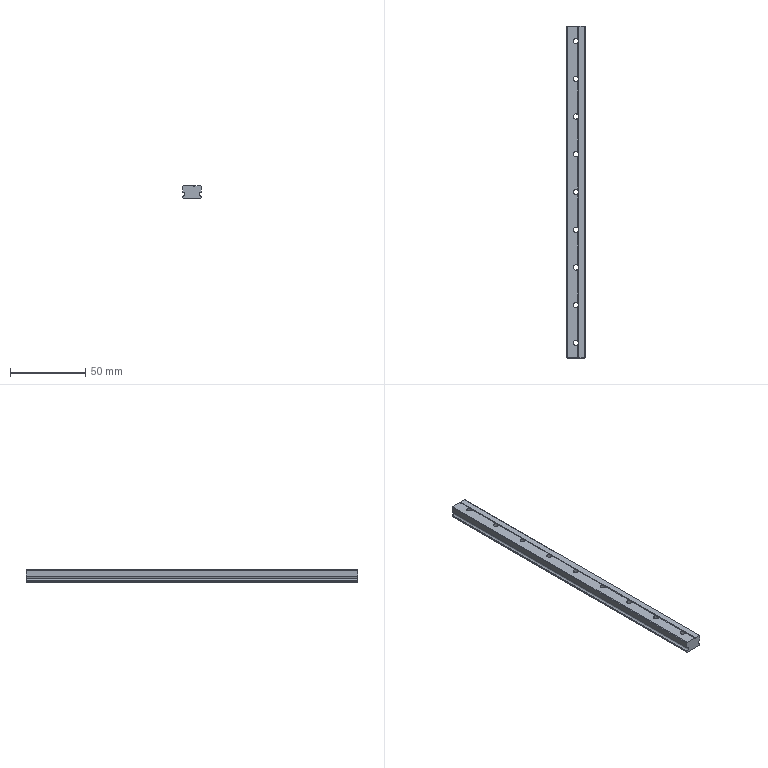Component | SolidWorks | LinearGuideMGN12(HIWIN)-1 | 1 solid | 169 faces | box 12 x 220 x 8 mm | volume 18690 mm3 | plane 114 | cylinder 40 | spline 15 | commonest cylinder face diameters 6 x18 3.5 x18 2.5 x3 0.6 x1 | material Chrome Stainless Steel
build123d program:
from build123d import *

# Parameters (mm, degrees)
BOSS_EXTRUDE1_DEPTH                             = 220
M3_HEX_SOCKET_HEAD_CAP_SCREW_CBORE1_D           = 3.5
M3_HEX_SOCKET_HEAD_CAP_SCREW_CBORE1_CBORE_D     = 6
M3_HEX_SOCKET_HEAD_CAP_SCREW_CBORE1_CBORE_DEPTH = 3.5
LPATTERN1_COUNT                                 = 9
LPATTERN1_PITCH                                 = 25
SKETCH6_W                                       = 2
SKETCH6_H                                       = 0.1795
CUT_EXTRUDE1_DEPTH                              = 0.1


with BuildPart() as part:
    # Sketch1 → Boss-Extrude1 (new body)
    with BuildSketch(Plane.XY):
        with BuildLine():
            Line((-5.7, 0), (1.2, 0))
            ThreePointArc((1.2, 0), (1.5, 0.3), (1.8, 0))
            Line((1.8, 0), (5.7, 0))
            Line((5.7, 0), (6, 0.3))
            Line((6, 0.3), (6, 4.25))
            ThreePointArc((6, 4.25), (4.75, 5.5), (6, 6.75))
            Line((6, 6.75), (6, 7.7))
            Line((6, 7.7), (5.7, 8))
            Line((5.7, 8), (-5.7, 8))
            Line((-5.7, 8), (-6, 7.7))
            Line((-6, 7.7), (-6, 6.75))
            ThreePointArc((-6, 6.75), (-4.75, 5.5), (-6, 4.25))
            Line((-6, 4.25), (-6, 0.3))
            Line((-6, 0.3), (-5.7, 0))
        make_face()
    extrude(amount=-BOSS_EXTRUDE1_DEPTH)

    # M3 Hex Socket Head Cap Screw CBORE1 (through all)
    with Locations(Plane(origin=(1.75, 8, 16.517), x_dir=(-1, 0, 0), z_dir=(0, 1, 0))):
        with Locations((1.75, -26.517)):
            m3_hex_socket_head_cap_screw_cbore1 = CounterBoreHole(M3_HEX_SOCKET_HEAD_CAP_SCREW_CBORE1_D / 2, M3_HEX_SOCKET_HEAD_CAP_SCREW_CBORE1_CBORE_D / 2, M3_HEX_SOCKET_HEAD_CAP_SCREW_CBORE1_CBORE_DEPTH)

    # LPattern1: M3 Hex Socket Head Cap Screw CBORE1 ×9
    with Locations(*[(0, 0, -i * LPATTERN1_PITCH) for i in range(1, LPATTERN1_COUNT)]):
        add(m3_hex_socket_head_cap_screw_cbore1, mode=Mode.SUBTRACT)

    # Sketch6 → Cut-Extrude1 (cut)
    with BuildSketch(Plane(origin=(0, 8, 0), x_dir=(1, 0, 0), z_dir=(0, 1, 0))):
        Polygon((-2, 13.385), (-2, 13.564), (-1.179, 13.564), (-1.179, 14.59), (-2, 14.59), (-2, 14.769), (0, 14.769), (0, 14.59), (-0.9744, 14.59), (-0.9744, 13.564), (0, 13.564), (0, 13.385), align=None)
        with Locations((-1, 15.372)):
            Rectangle(SKETCH6_W, SKETCH6_H)
        Polygon((-2, 15.769), (-2, 15.955), (-0.5333, 16.346), (-2, 16.928), (-2, 16.954), (-0.5433, 17.526), (-2, 17.919), (-2, 18.103), (0, 17.563), (0, 17.538), (-1.53, 16.936), (0, 16.327), (0, 16.301), align=None)
        with Locations((-1, 18.654)):
            Rectangle(SKETCH6_W, SKETCH6_H)
        Polygon((0, 19.179), (-2, 19.179), (-2, 19.217), (-0.4259, 20.538), (-2, 20.538), (-2, 20.718), (0, 20.718), (0, 20.677), (-1.571, 19.359), (0, 19.359), align=None)
        Polygon((0, 21.897), (-2, 22.161), (-2, 22.187), (-0.359, 23.013), (-2, 23.837), (-2, 23.863), (0, 24.128), (0, 23.948), (-1.439, 23.756), (0, 23.034), (0, 22.994), (-1.442, 22.269), (0, 22.078), align=None)
        with BuildLine():
            Line((-1.659, 26.41), (-1.513, 26.256))
            add(Edge.make_bspline(
                [(-1.513, 26.256), (-1.539, 26.229), (-1.591, 26.174), (-1.658, 26.084), (-1.716, 25.99), (-1.763, 25.893), (-1.799, 25.795), (-1.826, 25.698), (-1.843, 25.601), (-1.845, 25.537), (-1.846, 25.506)],
                knots=[0, 0, 0, 0, 1.089, 2.152, 3.19, 4.218, 5.218, 6.174, 7.1, 8, 8, 8, 8], degree=3))
            add(Edge.make_bspline(
                [(-1.846, 25.506), (-1.846, 25.486), (-1.845, 25.448), (-1.839, 25.39), (-1.831, 25.333), (-1.818, 25.277), (-1.802, 25.221), (-1.782, 25.167), (-1.759, 25.112), (-1.732, 25.06), (-1.703, 25.008), (-1.67, 24.96), (-1.636, 24.914), (-1.598, 24.871), (-1.558, 24.832), (-1.515, 24.795), (-1.47, 24.761), (-1.423, 24.731), (-1.374, 24.704), (-1.323, 24.68), (-1.273, 24.66), (-1.221, 24.644), (-1.169, 24.631), (-1.116, 24.622), (-1.063, 24.617), (-1.027, 24.616), (-1.009, 24.615)],
                knots=[0, 0, 0, 0, 1.028, 2.054, 3.065, 4.081, 5.107, 6.131, 7.173, 8.228, 9.276, 10.308, 11.325, 12.329, 13.321, 14.316, 15.309, 16.309, 17.306, 18.285, 19.246, 20.203, 21.146, 22.095, 23.042, 24, 24, 24, 24], degree=3))
            add(Edge.make_bspline(
                [(-1.009, 24.615), (-0.9904, 24.616), (-0.9535, 24.617), (-0.8986, 24.622), (-0.8444, 24.632), (-0.791, 24.646), (-0.7382, 24.663), (-0.6861, 24.685), (-0.6347, 24.71), (-0.5846, 24.739), (-0.5357, 24.771), (-0.4893, 24.807), (-0.4459, 24.846), (-0.4048, 24.887), (-0.3664, 24.931), (-0.331, 24.979), (-0.2982, 25.03), (-0.2682, 25.083), (-0.2415, 25.138), (-0.2177, 25.195), (-0.1981, 25.253), (-0.1821, 25.313), (-0.169, 25.373), (-0.1606, 25.436), (-0.1545, 25.499), (-0.1541, 25.542), (-0.1538, 25.563)],
                knots=[0, 0, 0, 0, 0.9359, 1.869, 2.8, 3.73, 4.665, 5.616, 6.583, 7.57, 8.563, 9.553, 10.533, 11.515, 12.51, 13.508, 14.526, 15.561, 16.601, 17.643, 18.681, 19.72, 20.772, 21.833, 22.908, 24, 24, 24, 24], degree=3))
            add(Edge.make_bspline(
                [(-0.1538, 25.563), (-0.1544, 25.589), (-0.1555, 25.64), (-0.1637, 25.715), (-0.1767, 25.787), (-0.1957, 25.856), (-0.2197, 25.921), (-0.2494, 25.984), (-0.2845, 26.044), (-0.3243, 26.1), (-0.3686, 26.152), (-0.416, 26.199), (-0.4671, 26.239), (-0.5211, 26.275), (-0.5786, 26.305), (-0.6392, 26.329), (-0.7029, 26.347), (-0.747, 26.355), (-0.7692, 26.359)],
                knots=[0, 0, 0, 0, 1.13, 2.219, 3.279, 4.312, 5.323, 6.328, 7.327, 8.334, 9.329, 10.292, 11.241, 12.174, 13.112, 14.052, 15.016, 16, 16, 16, 16], degree=3))
            Line((-0.7692, 26.359), (-0.7692, 25.692))
            Line((-0.7692, 25.692), (-0.9744, 25.692))
            Line((-0.9744, 25.692), (-0.9744, 26.538))
            add(Edge.make_bspline(
                [(-0.9744, 26.538), (-0.9361, 26.537), (-0.8613, 26.536), (-0.7522, 26.522), (-0.6491, 26.501), (-0.552, 26.471), (-0.4609, 26.433), (-0.3759, 26.386), (-0.2974, 26.331), (-0.2248, 26.268), (-0.16, 26.198), (-0.1031, 26.122), (-0.05518, 26.04), (-0.01617, 25.953), (0.01427, 25.859), (0.03585, 25.76), (0.04878, 25.656), (0.05044, 25.584), (0.05128, 25.548)],
                knots=[0, 0, 0, 0, 1.14, 2.232, 3.274, 4.278, 5.255, 6.214, 7.164, 8.118, 9.068, 10.008, 10.945, 11.892, 12.865, 13.864, 14.908, 16, 16, 16, 16], degree=3))
            add(Edge.make_bspline(
                [(0.05128, 25.548), (0.05096, 25.525), (0.05032, 25.481), (0.04576, 25.415), (0.03874, 25.351), (0.02814, 25.289), (0.01516, 25.228), (-0.001459, 25.17), (-0.0207, 25.113), (-0.04258, 25.057), (-0.06794, 25.004), (-0.09611, 24.952), (-0.127, 24.903), (-0.161, 24.855), (-0.198, 24.808), (-0.2381, 24.764), (-0.2811, 24.721), (-0.3116, 24.695), (-0.3269, 24.681)],
                knots=[0, 0, 0, 0, 1.108, 2.185, 3.234, 4.263, 5.276, 6.27, 7.252, 8.226, 9.19, 10.146, 11.103, 12.066, 13.032, 14.011, 14.998, 16, 16, 16, 16], degree=3))
            add(Edge.make_bspline(
                [(-0.3269, 24.681), (-0.3513, 24.662), (-0.3997, 24.623), (-0.4772, 24.573), (-0.5574, 24.53), (-0.6406, 24.496), (-0.7267, 24.469), (-0.8155, 24.45), (-0.9073, 24.438), (-0.9694, 24.437), (-1.001, 24.436)],
                knots=[0, 0, 0, 0, 1.023, 2.029, 3.014, 3.995, 4.976, 5.966, 6.971, 8, 8, 8, 8], degree=3))
            add(Edge.make_bspline(
                [(-1.001, 24.436), (-1.024, 24.436), (-1.071, 24.437), (-1.14, 24.444), (-1.209, 24.455), (-1.276, 24.47), (-1.341, 24.49), (-1.406, 24.514), (-1.469, 24.542), (-1.53, 24.575), (-1.59, 24.612), (-1.646, 24.652), (-1.699, 24.695), (-1.749, 24.742), (-1.795, 24.791), (-1.838, 24.844), (-1.878, 24.9), (-1.914, 24.96), (-1.946, 25.022), (-1.974, 25.086), (-1.998, 25.152), (-2.018, 25.22), (-2.032, 25.29), (-2.043, 25.362), (-2.05, 25.436), (-2.051, 25.486), (-2.051, 25.512)],
                knots=[0, 0, 0, 0, 1.009, 2.005, 2.991, 3.967, 4.948, 5.927, 6.92, 7.92, 8.923, 9.906, 10.883, 11.852, 12.825, 13.799, 14.781, 15.774, 16.776, 17.772, 18.776, 19.79, 20.809, 21.852, 22.911, 24, 24, 24, 24], degree=3))
            add(Edge.make_bspline(
                [(-2.051, 25.512), (-2.051, 25.532), (-2.05, 25.573), (-2.046, 25.634), (-2.039, 25.695), (-2.029, 25.754), (-2.015, 25.812), (-1.999, 25.87), (-1.981, 25.926), (-1.958, 25.982), (-1.933, 26.037), (-1.905, 26.091), (-1.872, 26.145), (-1.837, 26.199), (-1.797, 26.253), (-1.754, 26.306), (-1.708, 26.359), (-1.675, 26.393), (-1.659, 26.41)],
                knots=[0, 0, 0, 0, 0.9859, 1.955, 2.915, 3.87, 4.815, 5.76, 6.705, 7.649, 8.608, 9.583, 10.581, 11.604, 12.66, 13.74, 14.853, 16, 16, 16, 16], degree=3))
        make_face()
        Polygon((0, 26.949), (-2, 26.949), (-2, 26.986), (-0.4259, 28.308), (-2, 28.308), (-2, 28.487), (0, 28.487), (0, 28.446), (-1.571, 27.128), (0, 27.128), align=None)
        Polygon((-2, 29.246), (-2, 29.615), (0, 29.615), (0, 29.436), (-1.795, 29.436), (-1.795, 29.128), align=None)
        with BuildLine():
            Line((-1.385, 30.615), (-1.385, 30.436))
            add(Edge.make_bspline(
                [(-1.385, 30.436), (-1.408, 30.437), (-1.455, 30.439), (-1.523, 30.45), (-1.589, 30.466), (-1.65, 30.487), (-1.709, 30.514), (-1.764, 30.547), (-1.816, 30.585), (-1.864, 30.629), (-1.908, 30.676), (-1.947, 30.727), (-1.979, 30.781), (-2.006, 30.837), (-2.026, 30.896), (-2.041, 30.957), (-2.05, 31.022), (-2.051, 31.066), (-2.051, 31.088)],
                knots=[0, 0, 0, 0, 1.101, 2.162, 3.184, 4.19, 5.176, 6.163, 7.152, 8.156, 9.156, 10.134, 11.092, 12.041, 13.001, 13.972, 14.969, 16, 16, 16, 16], degree=3))
            add(Edge.make_bspline(
                [(-2.051, 31.088), (-2.051, 31.11), (-2.05, 31.153), (-2.041, 31.216), (-2.028, 31.276), (-2.008, 31.332), (-1.983, 31.386), (-1.952, 31.436), (-1.917, 31.483), (-1.875, 31.526), (-1.83, 31.565), (-1.782, 31.599), (-1.733, 31.628), (-1.682, 31.652), (-1.628, 31.67), (-1.573, 31.683), (-1.515, 31.691), (-1.477, 31.692), (-1.457, 31.692)],
                knots=[0, 0, 0, 0, 1.112, 2.184, 3.213, 4.224, 5.211, 6.196, 7.192, 8.207, 9.22, 10.201, 11.166, 12.121, 13.065, 14.026, 14.997, 16, 16, 16, 16], degree=3))
            add(Edge.make_bspline(
                [(-1.457, 31.692), (-1.429, 31.691), (-1.374, 31.689), (-1.293, 31.673), (-1.214, 31.647), (-1.151, 31.617), (-1.1, 31.585), (-1.058, 31.557), (-1.012, 31.524), (-0.9638, 31.487), (-0.9124, 31.444), (-0.8573, 31.396), (-0.7993, 31.344), (-0.7597, 31.307), (-0.7392, 31.288)],
                knots=[0, 0, 0, 0, 1.184, 2.348, 3.509, 4.696, 5.334, 6.051, 6.844, 7.715, 8.667, 9.695, 10.806, 12, 12, 12, 12], degree=3))
            Line((-0.7392, 31.288), (-0.2051, 30.787))
            Line((-0.2051, 30.787), (-0.2051, 31.718))
            Line((-0.2051, 31.718), (0, 31.718))
            Line((0, 31.718), (0, 30.359))
            Line((0, 30.359), (-0.8277, 31.135))
            add(Edge.make_bspline(
                [(-0.8277, 31.135), (-0.8474, 31.153), (-0.8853, 31.19), (-0.9406, 31.241), (-0.9919, 31.287), (-1.039, 31.328), (-1.083, 31.364), (-1.122, 31.395), (-1.158, 31.42), (-1.199, 31.447), (-1.25, 31.474), (-1.312, 31.496), (-1.376, 31.51), (-1.419, 31.512), (-1.441, 31.513)],
                knots=[0, 0, 0, 0, 1.33, 2.554, 3.673, 4.688, 5.603, 6.414, 7.123, 7.735, 8.834, 9.9, 10.944, 12, 12, 12, 12], degree=3))
            add(Edge.make_bspline(
                [(-1.441, 31.513), (-1.454, 31.512), (-1.481, 31.512), (-1.521, 31.505), (-1.559, 31.496), (-1.595, 31.482), (-1.631, 31.464), (-1.664, 31.442), (-1.696, 31.417), (-1.727, 31.387), (-1.755, 31.355), (-1.779, 31.321), (-1.8, 31.285), (-1.817, 31.247), (-1.83, 31.208), (-1.839, 31.166), (-1.845, 31.123), (-1.846, 31.094), (-1.846, 31.079)],
                knots=[0, 0, 0, 0, 0.9914, 1.954, 2.896, 3.839, 4.798, 5.76, 6.748, 7.785, 8.825, 9.84, 10.836, 11.836, 12.849, 13.864, 14.912, 16, 16, 16, 16], degree=3))
            add(Edge.make_bspline(
                [(-1.846, 31.079), (-1.846, 31.063), (-1.845, 31.033), (-1.839, 30.988), (-1.83, 30.944), (-1.816, 30.903), (-1.8, 30.864), (-1.779, 30.827), (-1.754, 30.792), (-1.726, 30.759), (-1.694, 30.729), (-1.658, 30.703), (-1.62, 30.68), (-1.579, 30.659), (-1.535, 30.643), (-1.487, 30.63), (-1.437, 30.62), (-1.402, 30.617), (-1.385, 30.615)],
                knots=[0, 0, 0, 0, 1.031, 2.024, 2.988, 3.934, 4.865, 5.795, 6.73, 7.685, 8.651, 9.612, 10.592, 11.592, 12.625, 13.701, 14.822, 16, 16, 16, 16], degree=3))
        make_face()
    extrude(amount=-CUT_EXTRUDE1_DEPTH, mode=Mode.SUBTRACT)


solid = part.part

# Placed as in the assembly
solid = solid.moved(Location((-100.094, 103.23, 295), (-90, 0, 0)))